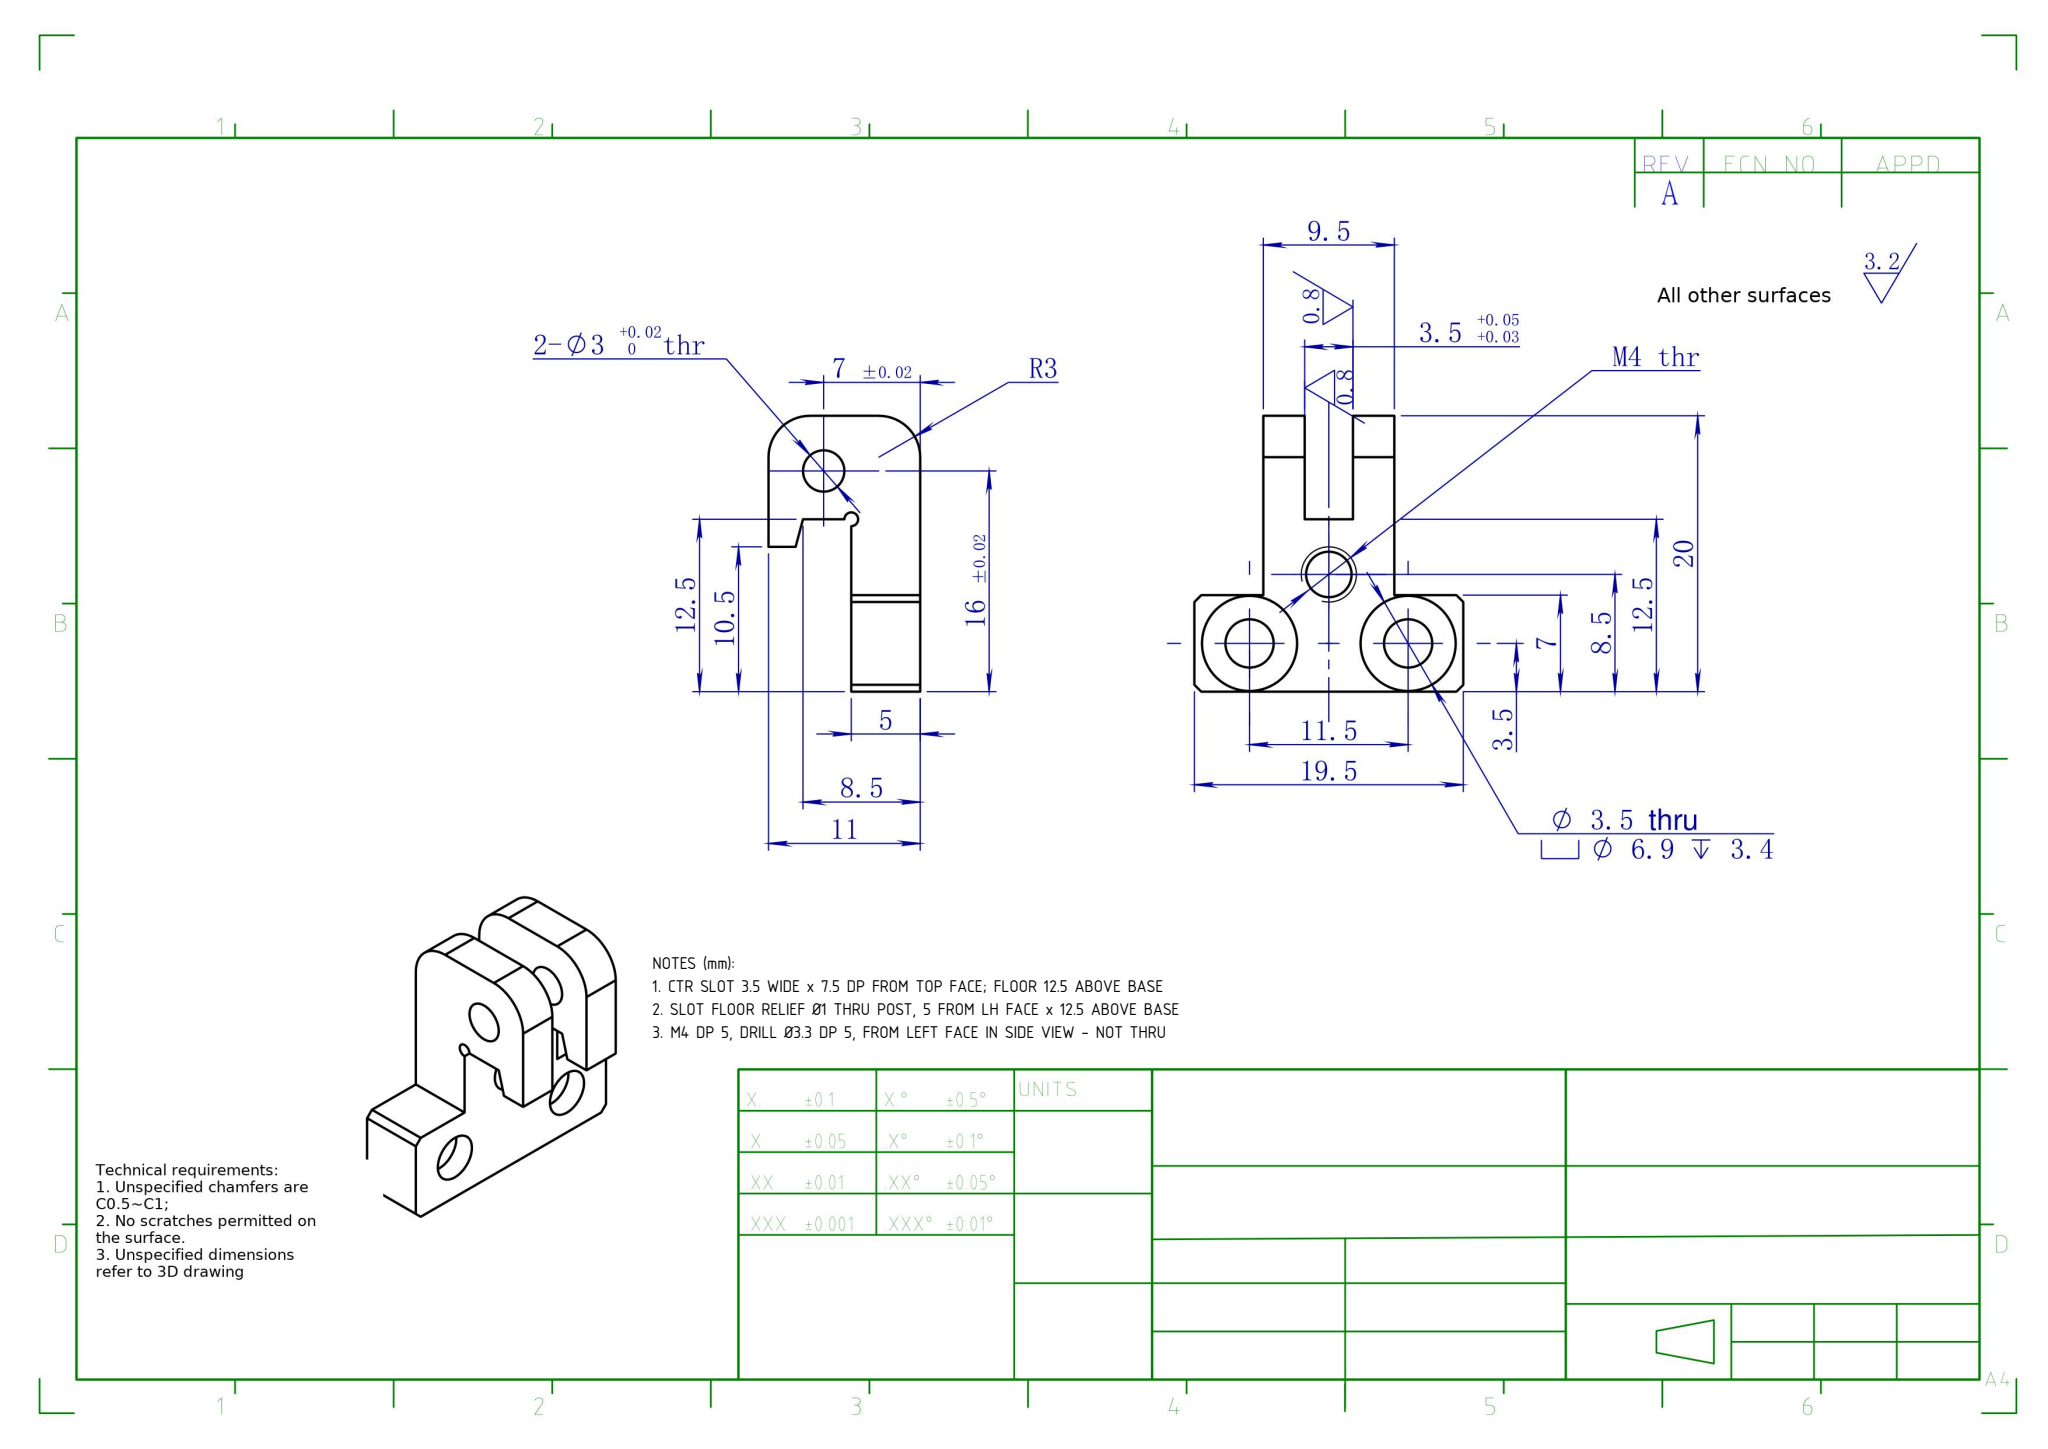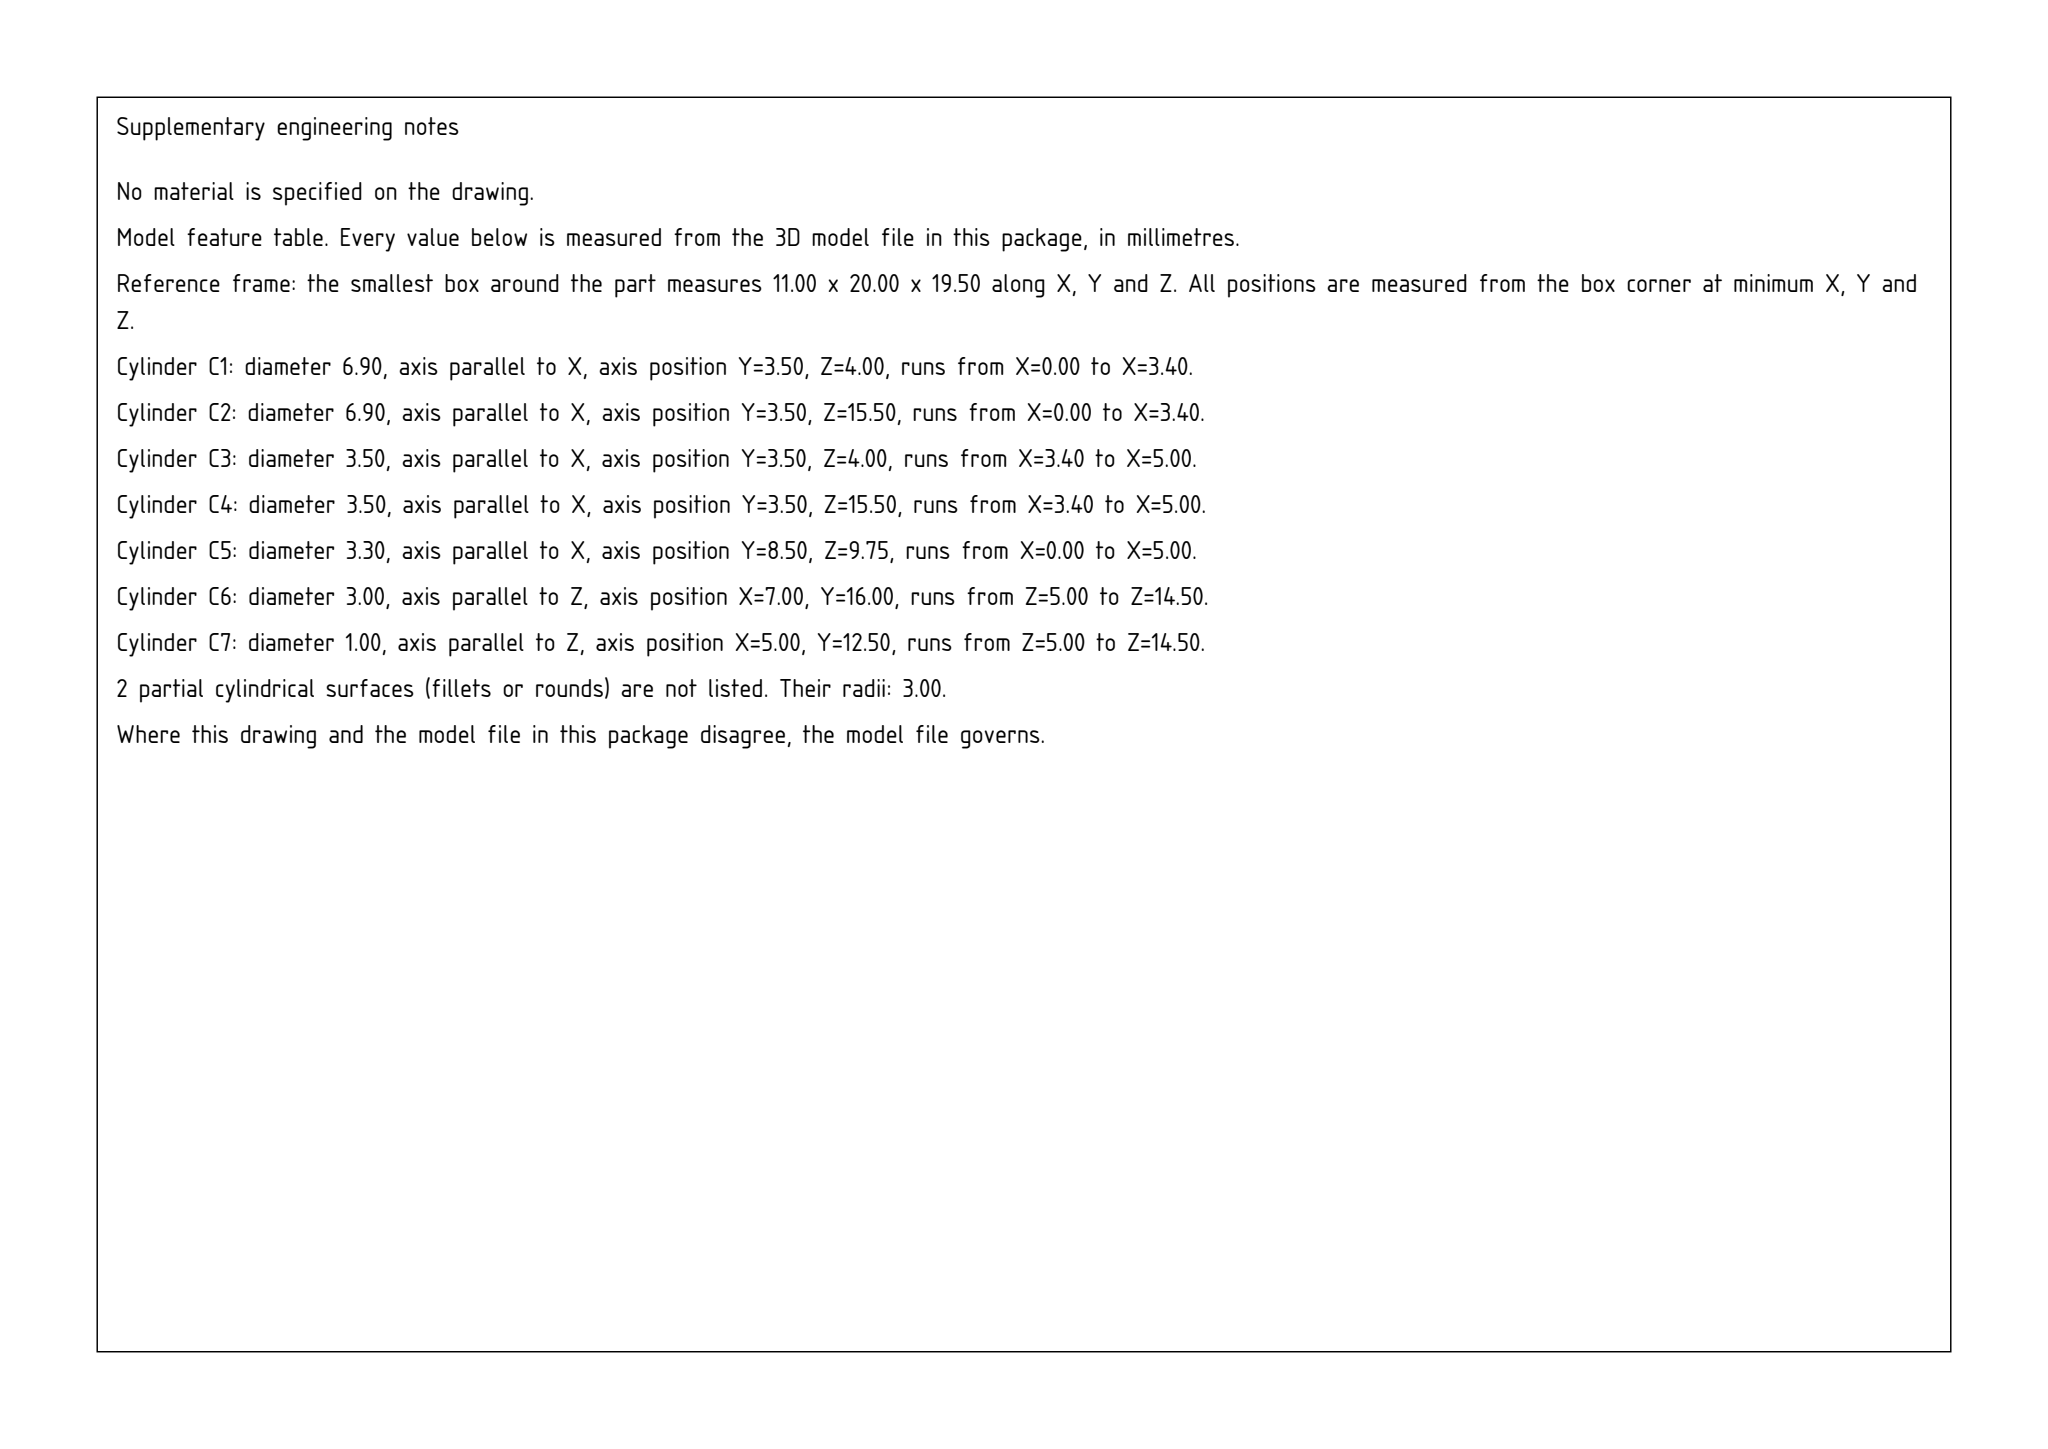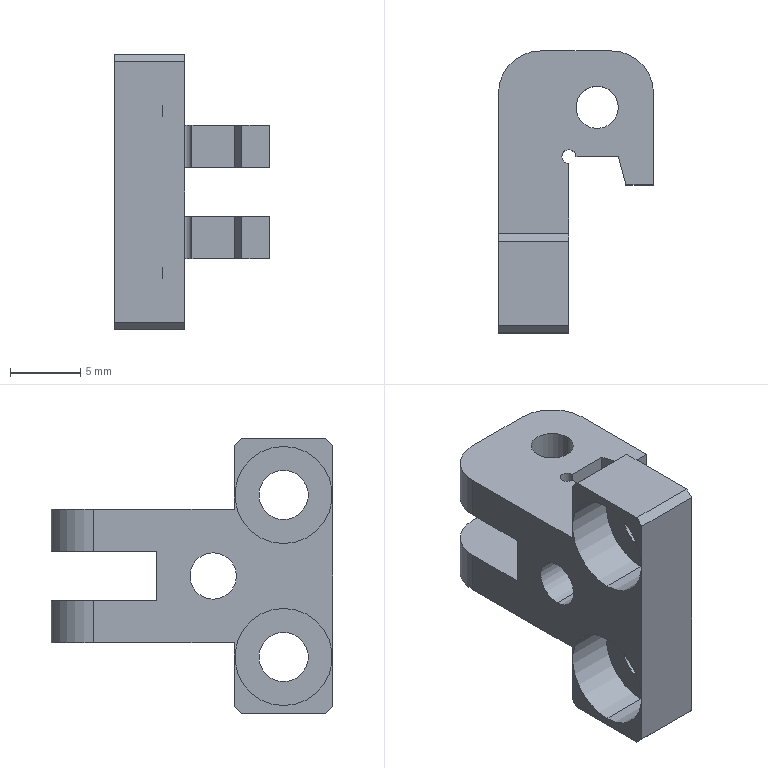Part | SolidWorks | mm | 1 solid | 49 faces | box 11 x 20 x 19.5 mm | volume 1065 mm3 | plane 28 | cylinder 21 | commonest cylinder face diameters 6.9 x4 3.5 x4 3 x4 6 x4 1 x3 3.3 x2
Drawing notes:
CTR SLOT 3.5 WIDE x 7.5 DP FROM TOP FACE; FLOOR 12.5 ABOVE BASE | from the solid: Slot flanks z=8.0 & 11.5 (3.5 wide) in 9.5 boss (z=5.0-14.5); floor plane y=12.5, top face y=20.0 -> 7.5 DP
SLOT FLOOR RELIEF Ø1 THRU POST, 5 FROM LH FACE x 12.5 ABOVE BASE | from the solid: cylinder dia 1.0, axis z, pos (5.0,12.5), length 9.5 = full post width
M4 DP 5, DRILL Ø3.3 DP 5, FROM LEFT FACE IN SIDE VIEW - NOT THRU | from the solid: cylinder [3.3, x-axis, y=8.5, z=9.75, length 5.0] starting at x=0 face; bbox x length 11.0 so hole is blind, not thru
build123d program:
from build123d import *

# Parameters (mm, degrees)
SKETCH1_W                                            = 11
SKETCH1_H                                            = 20
BOSS_EXTRUDE1_DEPTH                                  = 4.75
SKETCH2_W                                            = 6
SKETCH2_H                                            = 12.5
CUT_EXTRUDE1_DEPTH                                   = 15.849
SKETCH3_W                                            = 3.5
SKETCH3_H                                            = 7.5
CUT_EXTRUDE2_DEPTH                                   = 16.606
SKETCH4_R                                            = 1.5
CUT_EXTRUDE3_DEPTH                                   = 15.849
FILLET1_R                                            = 3
SKETCH5_R                                            = 1.5
CUT_EXTRUDE4_DEPTH                                   = 10
SKETCH6_W                                            = 5
SKETCH6_H                                            = 7
BOSS_EXTRUDE2_DEPTH                                  = 5
SKETCH7_W                                            = 2.5
SKETCH7_H                                            = 3
BOSS_EXTRUDE3_DEPTH                                  = 2
CUT_EXTRUDE5_DEPTH                                   = 19.453
COUNTERBORE_FOR_M3_HEX_SOCKET_HEAD_CAP_S_D           = 3.5
COUNTERBORE_FOR_M3_HEX_SOCKET_HEAD_CAP_S_CBORE_D     = 6.9
COUNTERBORE_FOR_M3_HEX_SOCKET_HEAD_CAP_S_CBORE_DEPTH = 3.4
CHAMFER1_SIZE                                        = 0.5
M4_TAPPED_HOLE1_D                                    = 3.3
M4_TAPPED_HOLE1_DEPTH                                = 11.5
M4_TAPPED_HOLE1_TIP                                  = 0.9914
SKETCH13_R                                           = 0.5
CUT_EXTRUDE6_DEPTH                                   = 19.453


with BuildPart() as part:
    # Sketch1 → Boss-Extrude1 (new, symmetric)
    with BuildSketch(Plane.XY):
        Rectangle(SKETCH1_W, SKETCH1_H)
    extrude(amount=BOSS_EXTRUDE1_DEPTH, both=True)

    # Sketch2 → Cut-Extrude1 (cut, through all)
    with BuildSketch(Plane.XY.offset(4.75)):
        with Locations((2.5, -3.75)):
            Rectangle(SKETCH2_W, SKETCH2_H)
    extrude(amount=-CUT_EXTRUDE1_DEPTH, mode=Mode.SUBTRACT)

    # Sketch3 → Cut-Extrude2 (cut, through all)
    with BuildSketch(Plane.ZY.offset(5.5)):
        with Locations((0, 6.25)):
            Rectangle(SKETCH3_W, SKETCH3_H)
    extrude(amount=-CUT_EXTRUDE2_DEPTH, mode=Mode.SUBTRACT)

    # Sketch4 → Cut-Extrude3 (cut, through all)
    with BuildSketch(Plane.XY.offset(4.75)):
        with Locations((1.5, 6)):
            Circle(SKETCH4_R)
    extrude(amount=-CUT_EXTRUDE3_DEPTH, mode=Mode.SUBTRACT)

    # Fillet1
    fillet1_edges = [part.edges().sort_by_distance(p)[0] for p in [
        (-5.5, 10, -3.25),
        (5.5, 10, -3.25),
        (-5.5, 10, 3.25),
        (5.5, 10, 3.25),
    ]]
    fillet(fillet1_edges, radius=FILLET1_R)

    # Sketch5 → Cut-Extrude4 (cut)
    with BuildSketch(Plane.ZY.offset(5.5)):
        with Locations(Location((0, -1.5, 0), (0, 0, 270))):
            Circle(SKETCH5_R)
    extrude(amount=-CUT_EXTRUDE4_DEPTH, mode=Mode.SUBTRACT)

    # Sketch6 → Boss-Extrude2 (add)
    with BuildSketch(Plane.XY.offset(4.75)):
        with Locations((-3, -6.5)):
            Rectangle(SKETCH6_W, SKETCH6_H)
    boss_extrude2 = extrude(amount=BOSS_EXTRUDE2_DEPTH)

    # Mirror1: Boss-Extrude2 across plane
    add(boss_extrude2.mirror(Plane.XY))

    # Sketch7 → Boss-Extrude3 (add)
    with BuildSketch(Plane.XZ.offset(-2.5)):
        with Locations((4.25, 3.25)):
            Rectangle(SKETCH7_W, SKETCH7_H)
    boss_extrude3 = extrude(amount=BOSS_EXTRUDE3_DEPTH)

    # Sketch8 → Cut-Extrude5 (cut, through all)
    with BuildSketch(Plane.XY.offset(4.75)):
        Polygon((3, 2.5), (3.536, 0.5), (3, 0.5), align=None)
    cut_extrude5 = extrude(amount=-CUT_EXTRUDE5_DEPTH, mode=Mode.SUBTRACT)

    # Mirror2: Boss-Extrude3, Cut-Extrude5 across plane
    add(boss_extrude3.mirror(Plane.XY))
    add(cut_extrude5.mirror(Plane.XY), mode=Mode.SUBTRACT)

    # Counterbore for M3 Hex Socket Head Cap S (through all)
    with Locations(Plane.ZY.offset(5.5)):
        with Locations((-5.75, -6.5)):
            counterbore_for_m3_hex_socket_head_cap_s = CounterBoreHole(COUNTERBORE_FOR_M3_HEX_SOCKET_HEAD_CAP_S_D / 2, COUNTERBORE_FOR_M3_HEX_SOCKET_HEAD_CAP_S_CBORE_D / 2, COUNTERBORE_FOR_M3_HEX_SOCKET_HEAD_CAP_S_CBORE_DEPTH)

    # Mirror3: Counterbore for M3 Hex Socket Head Cap S across plane
    add(counterbore_for_m3_hex_socket_head_cap_s.mirror(Plane.XY), mode=Mode.SUBTRACT)

    # Chamfer1
    chamfer1_edges = [part.edges().sort_by_distance(p)[0] for p in [
        (-3, -10, 9.75),
        (-3, -10, -9.75),
        (-3, -3, -9.75),
        (-3, -3, 9.75),
    ]]
    chamfer(chamfer1_edges, length=CHAMFER1_SIZE)

    # M4 Tapped Hole1
    with Locations(Plane.ZY.offset(5.5)):
        with Locations((0, -1.5)):
            Hole(M4_TAPPED_HOLE1_D / 2, depth=M4_TAPPED_HOLE1_DEPTH)
            with Locations((0, 0, -(M4_TAPPED_HOLE1_DEPTH + M4_TAPPED_HOLE1_TIP / 2))):  # 118° drill point
                Cone(0, M4_TAPPED_HOLE1_D / 2, M4_TAPPED_HOLE1_TIP, mode=Mode.SUBTRACT)

    # Sketch13 → Cut-Extrude6 (cut, through all)
    with BuildSketch(Plane(origin=(0, 0, -4.75), x_dir=(-1, 0, 0), z_dir=(0, 0, -1))):
        with Locations((0.5, 2.5)):
            Circle(SKETCH13_R)
    extrude(amount=-CUT_EXTRUDE6_DEPTH, mode=Mode.SUBTRACT)


solid = part.part